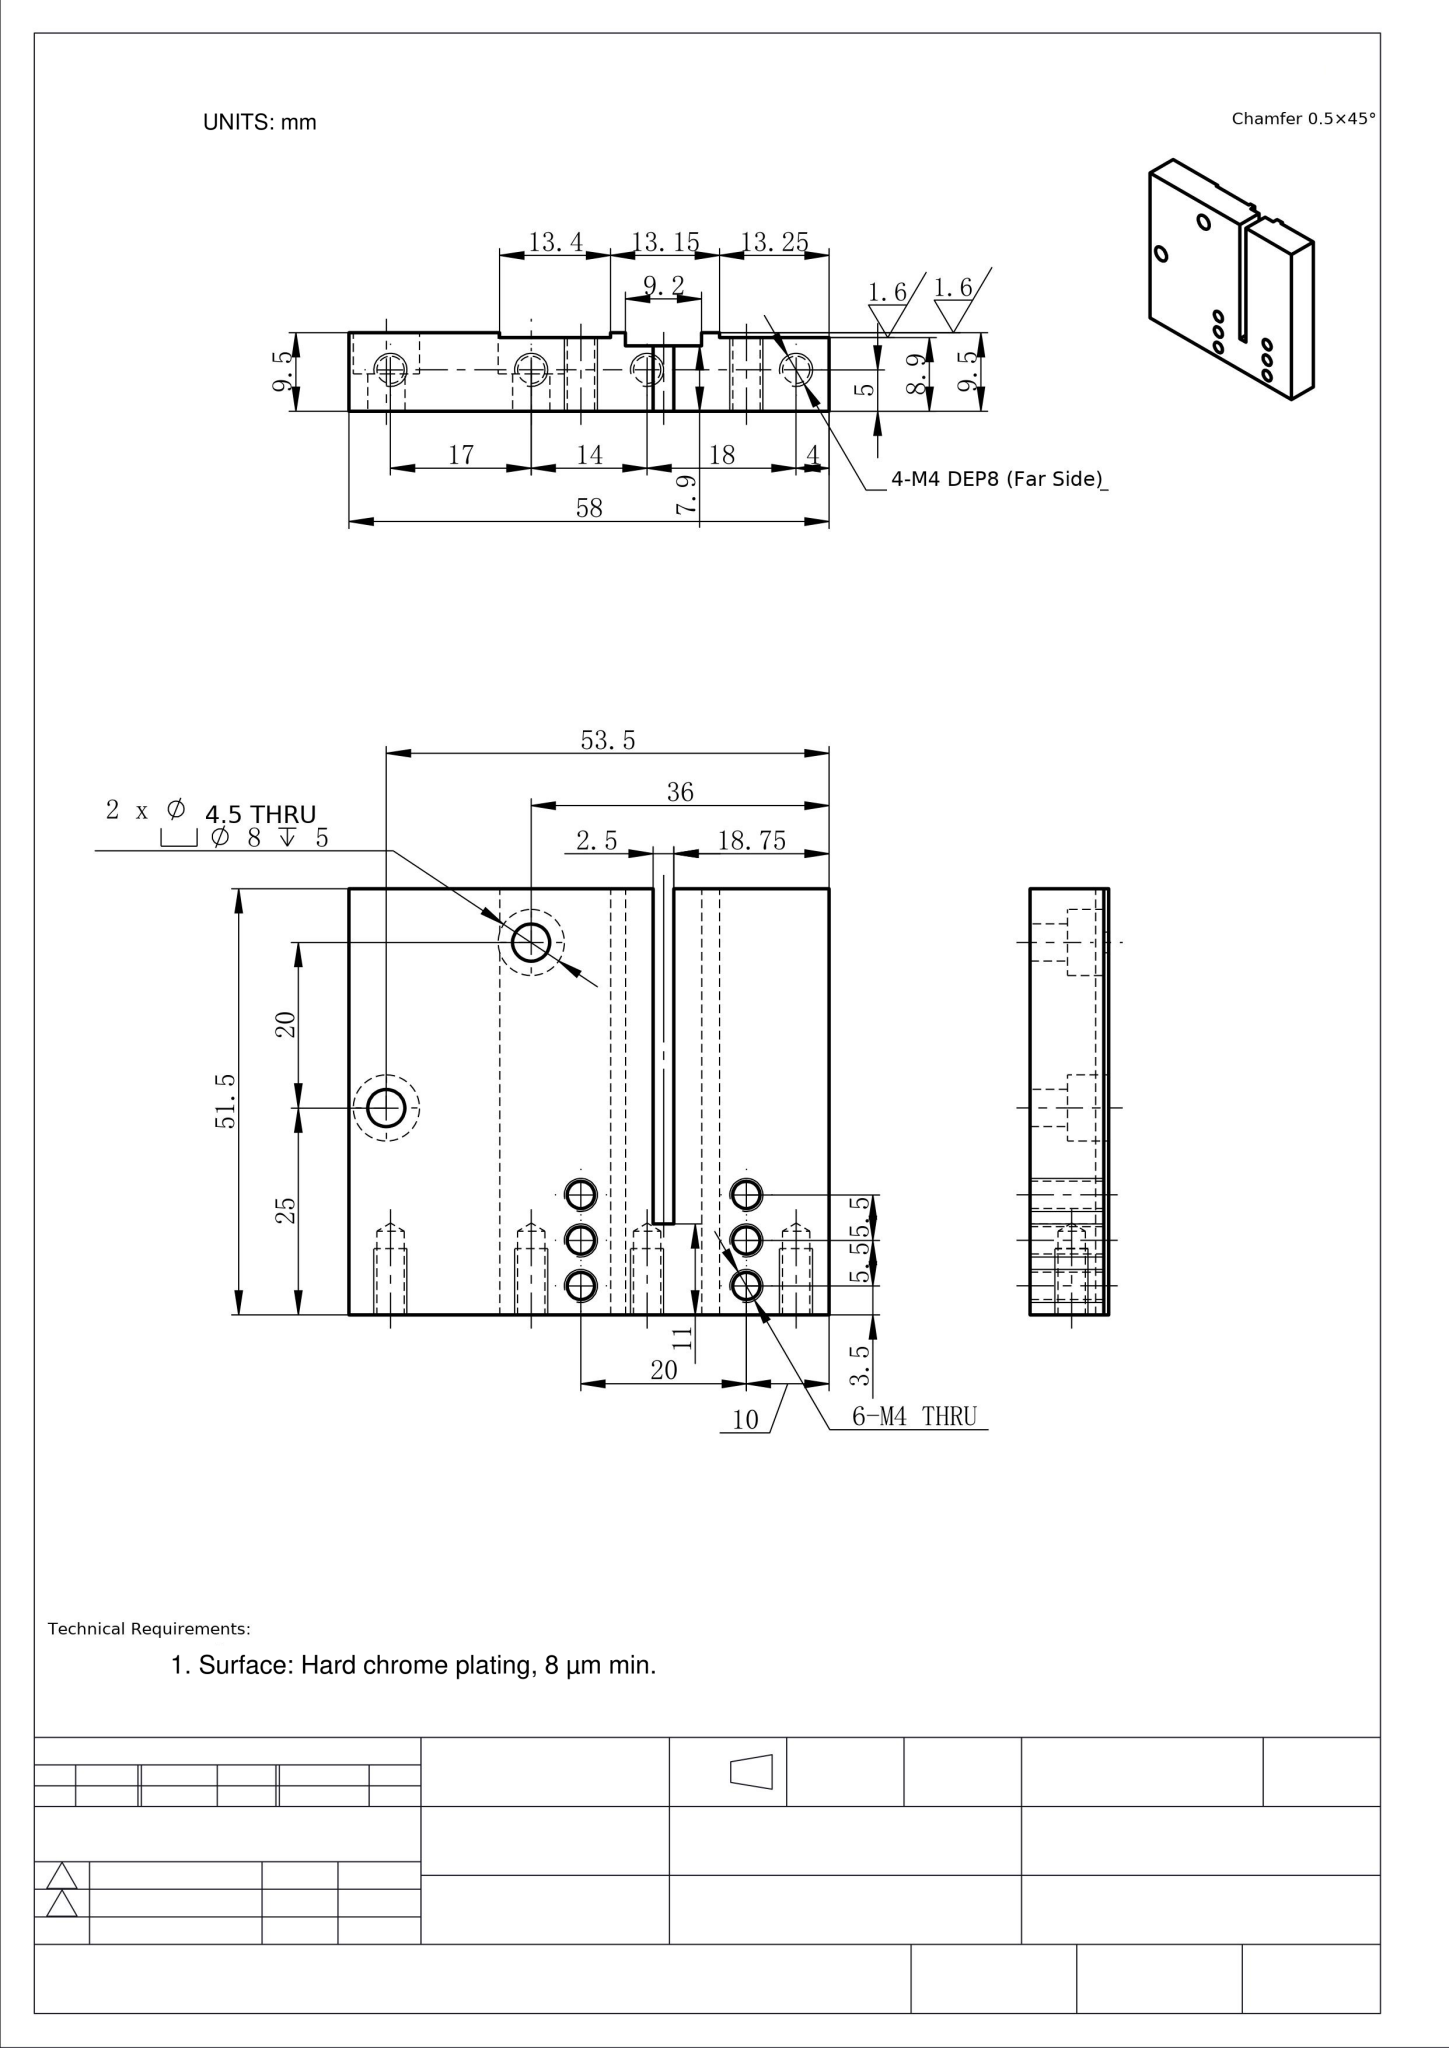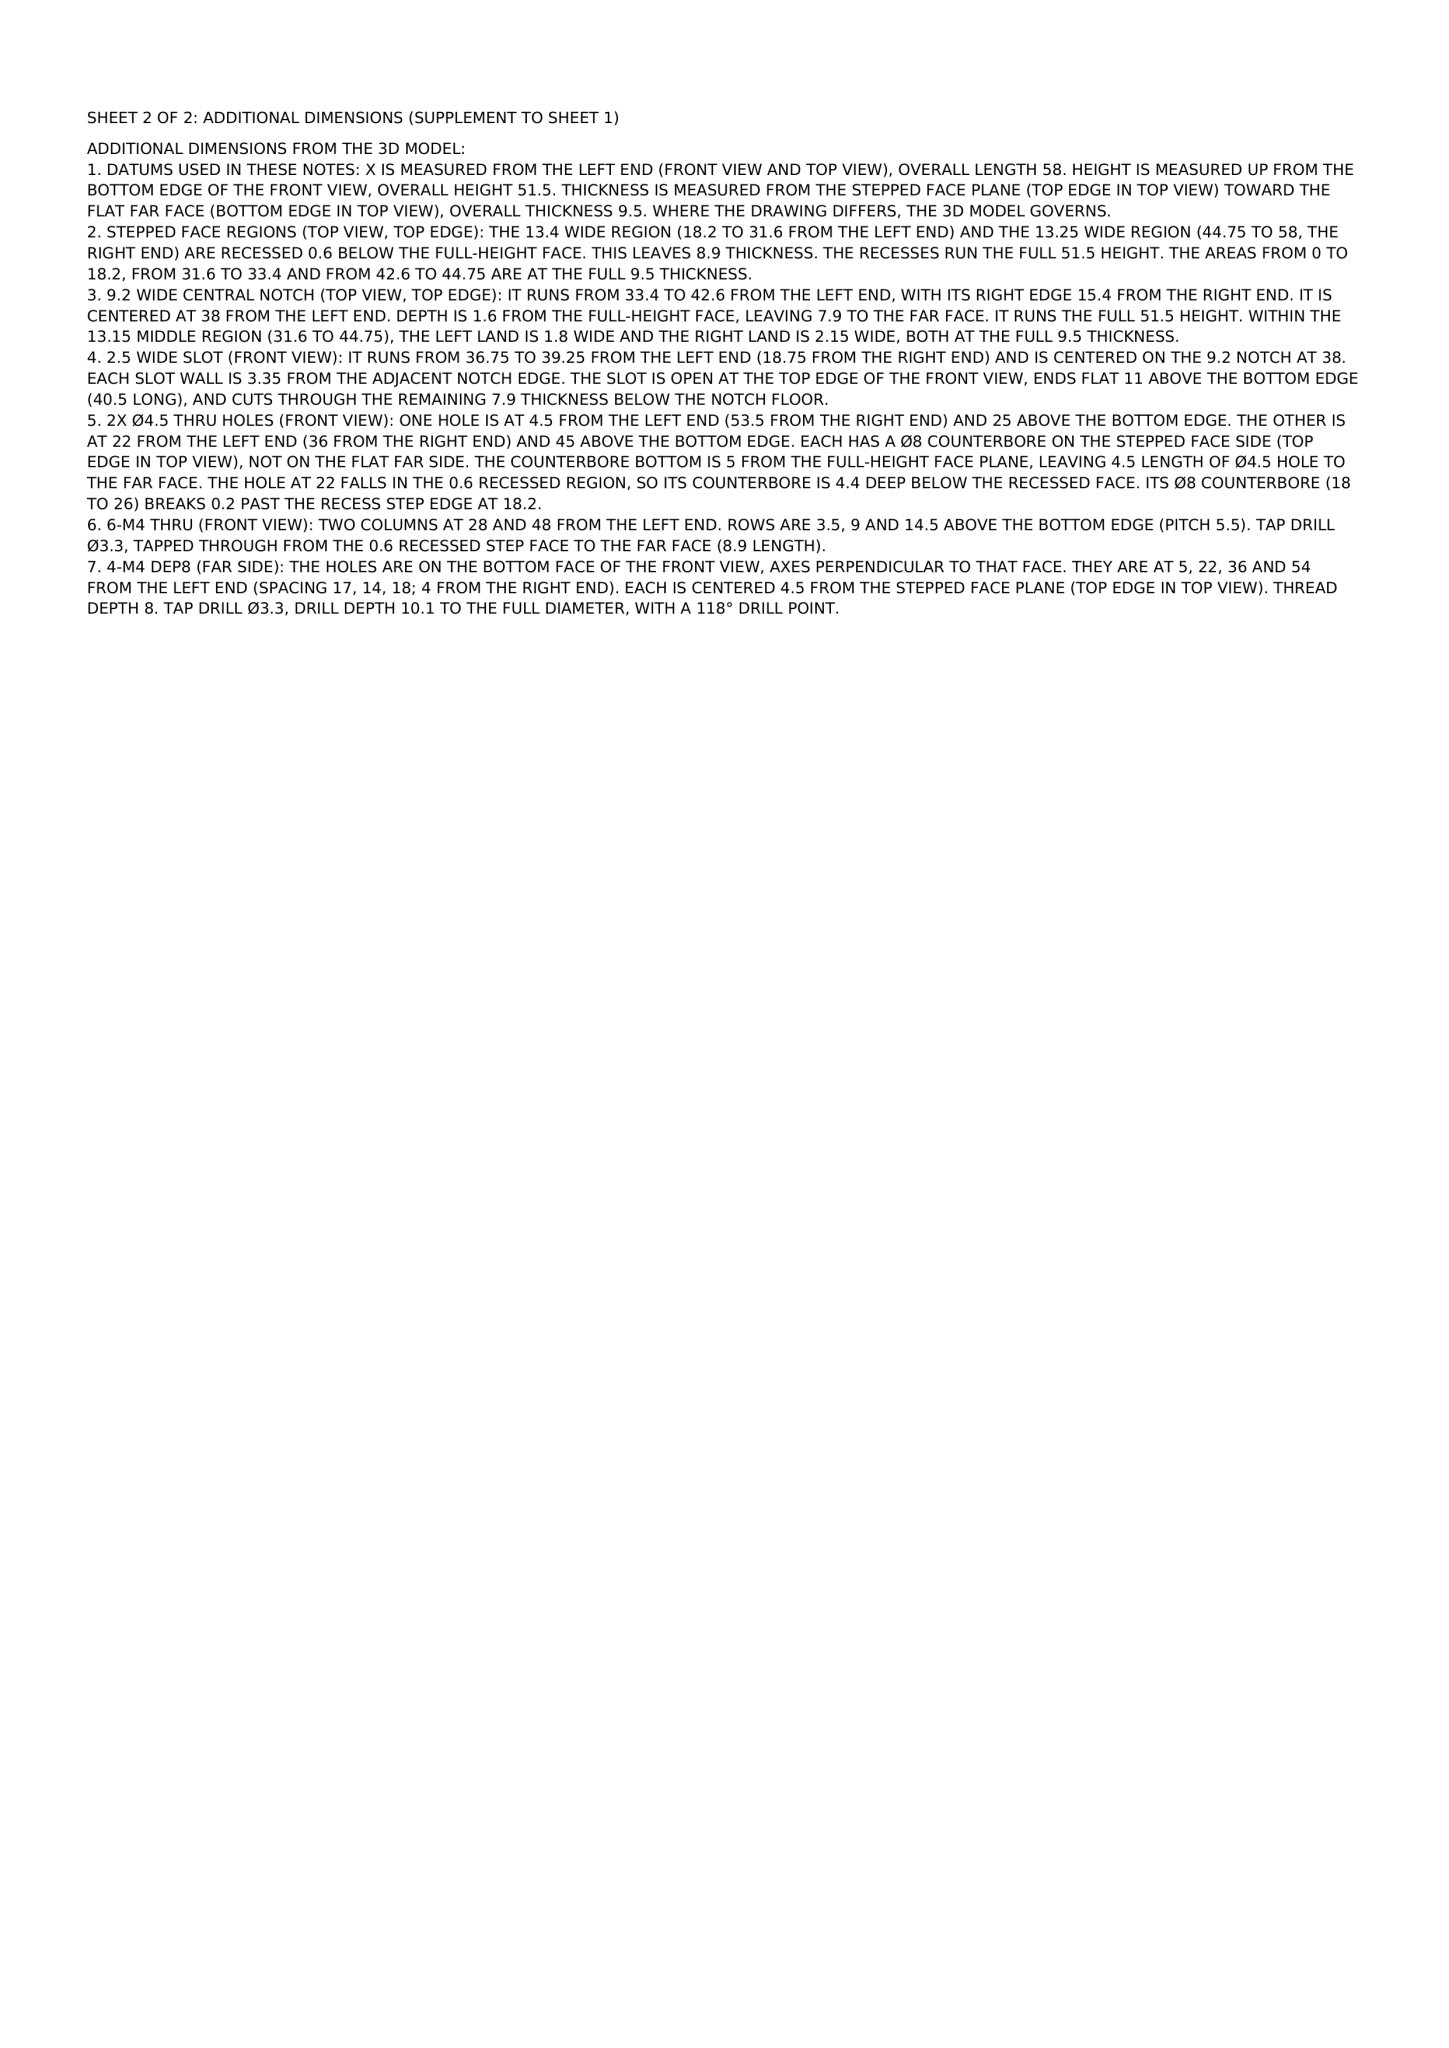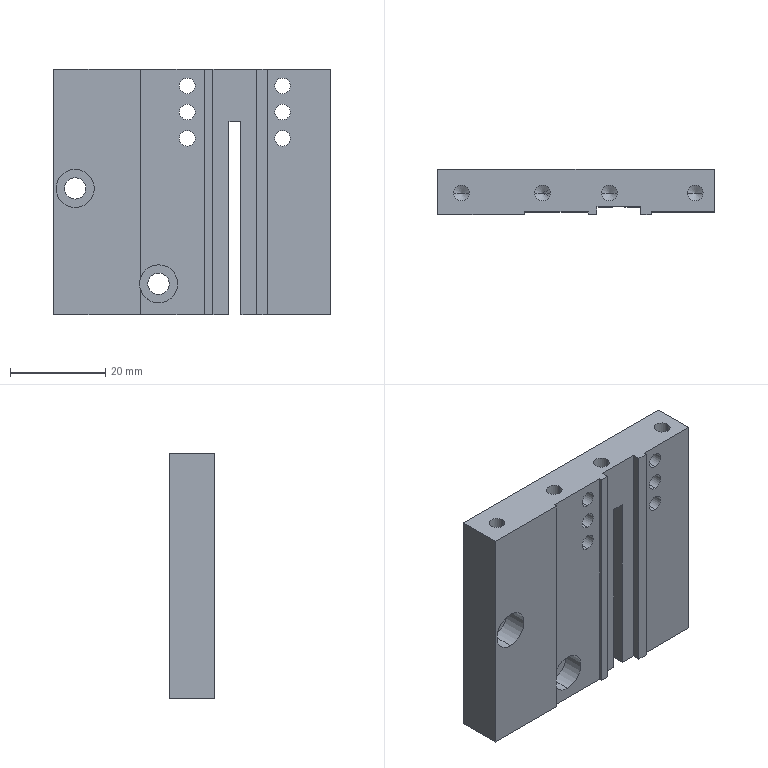Part | NX | mm | 1 solid | 59 faces | box 58 x 9.5 x 51.5 mm | volume 24566 mm3 | cylinder 28 | plane 23 | cone 8 | commonest cylinder face diameters 3.3 x20 8 x4 4.5 x4